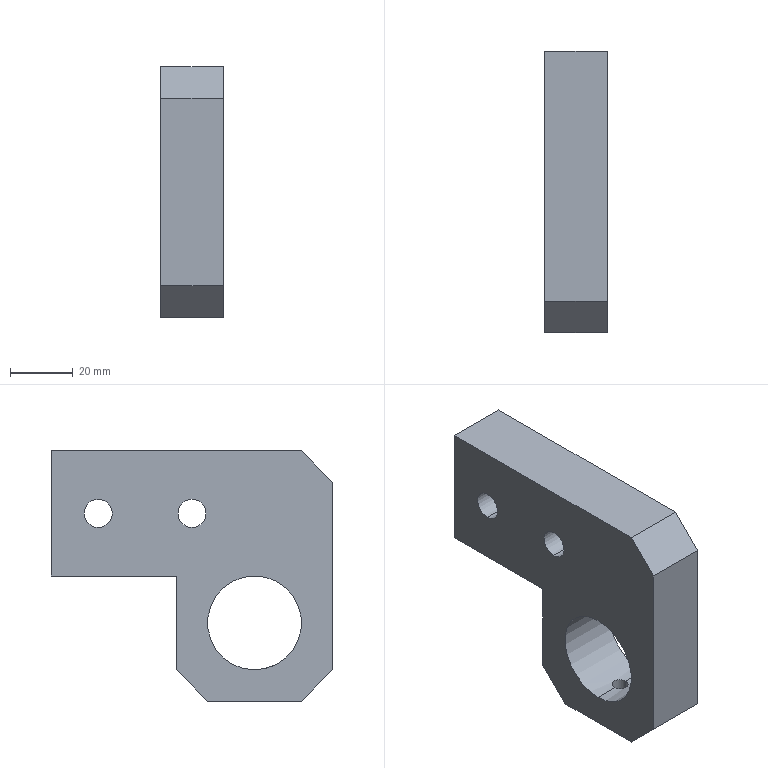Component | SolidWorks | UpperAxisBracket-1 | 1 solid | 19 faces | box 20 x 90 x 80 mm | volume 92121 mm3 | plane 11 | cylinder 8 | commonest cylinder face diameters 9 x4 5 x2 30 x2
build123d program:
from build123d import *

# Parameters (mm, degrees)
SKETCH1_R              = 15
BOSS_EXTRUDE1_DEPTH    = 20
SKETCH2_R              = 4.5
CUT_EXTRUDE1_DEPTH     = 123.066
CHAMFER1_SIZE          = 10
M6_TAPPED_HOLE1_REACH  = 124.066
M6_TAPPED_HOLE1_BORE_R = 2.5


with BuildPart() as part:
    # Sketch1 → Boss-Extrude1 (new body)
    with BuildSketch(Plane.XY):
        Polygon((0, 0), (0, 90), (80, 90), (80, 40), (40, 40), (40, 0), align=None)
        with Locations((55, 65)):
            Circle(SKETCH1_R, mode=Mode.SUBTRACT)
    extrude(amount=BOSS_EXTRUDE1_DEPTH)

    # Sketch2 → Cut-Extrude1 (cut, through all)
    with BuildSketch(Plane(origin=(0, 0, 0), x_dir=(-1, 0, 0), z_dir=(0, 0, -1))):
        with Locations((-20, 45)):
            Circle(SKETCH2_R)
        with Locations((-20, 15)):
            Circle(SKETCH2_R)
    extrude(amount=-CUT_EXTRUDE1_DEPTH, mode=Mode.SUBTRACT)

    # Chamfer1
    chamfer1_edges = [part.edges().sort_by_distance(p)[0] for p in [
        (0, 90, 10),
        (80, 90, 10),
        (80, 40, 10),
    ]]
    chamfer(chamfer1_edges, length=CHAMFER1_SIZE)

    # M6 Tapped Hole1 bore → M6 Tapped Hole1 (cut, up to next)
    with BuildSketch(Plane(origin=(80, 0, 0), x_dir=(0, 0, -1), z_dir=(1, 0, 0)), mode=Mode.PRIVATE) as m6_tapped_hole1_sk1:
        with Locations((-10, 65)):
            Circle(M6_TAPPED_HOLE1_BORE_R)
    m6_tapped_hole1_tool1 = extrude(m6_tapped_hole1_sk1.sketch, amount=-M6_TAPPED_HOLE1_REACH, mode=Mode.PRIVATE) & part.part
    add(m6_tapped_hole1_tool1.solids().sort_by_distance((80, 65, 10))[0], mode=Mode.SUBTRACT)


solid = part.part

# Placed as in the assembly
solid = solid.moved(Location((-5.532, -245.334, 1376.399), (180, -90, 0)))
STEP:
#1=COLOUR_RGB('',0.7922,0.8196,0.9333);
#2=FILL_AREA_STYLE_COLOUR('',#1);
#3=FILL_AREA_STYLE('',(#2));
#4=SURFACE_STYLE_FILL_AREA(#3);
#5=SURFACE_SIDE_STYLE('',(#4));
#6=SURFACE_STYLE_USAGE(.BOTH.,#5);
#7=PRESENTATION_STYLE_ASSIGNMENT((#6));
#8=CARTESIAN_POINT('',(-0.5131,-12.218,51.433));
#9=VERTEX_POINT('',#8);
#10=CARTESIAN_POINT('',(-0.7099,-12.218,51.433));
#11=VERTEX_POINT('',#10);
#12=CARTESIAN_POINT('',(-0.5131,-12.218,51.433));
#13=CARTESIAN_POINT('',(-0.5131,-12.211,51.433));
#14=CARTESIAN_POINT('',(-0.5137,-12.205,51.433));
#15=CARTESIAN_POINT('',(-0.5162,-12.192,51.434));
#16=CARTESIAN_POINT('',(-0.5181,-12.186,51.434));
#17=CARTESIAN_POINT('',(-0.5231,-12.174,51.435));
#18=CARTESIAN_POINT('',(-0.5261,-12.169,51.435));
#19=CARTESIAN_POINT('',(-0.5332,-12.158,51.436));
#20=CARTESIAN_POINT('',(-0.5374,-12.153,51.437));
#21=CARTESIAN_POINT('',(-0.551,-12.139,51.438));
#22=CARTESIAN_POINT('',(-0.5619,-12.132,51.439));
#23=CARTESIAN_POINT('',(-0.5797,-12.125,51.44));
#24=CARTESIAN_POINT('',(-0.5859,-12.123,51.441));
#25=CARTESIAN_POINT('',(-0.5986,-12.12,51.441));
#26=CARTESIAN_POINT('',(-0.605,-12.119,51.441));
#27=CARTESIAN_POINT('',(-0.6179,-12.119,51.441));
#28=CARTESIAN_POINT('',(-0.6244,-12.12,51.441));
#29=CARTESIAN_POINT('',(-0.637,-12.123,51.441));
#30=CARTESIAN_POINT('',(-0.6432,-12.124,51.44));
#31=CARTESIAN_POINT('',(-0.6551,-12.129,51.44));
#32=CARTESIAN_POINT('',(-0.6609,-12.132,51.439));
#33=CARTESIAN_POINT('',(-0.6715,-12.14,51.438));
#34=CARTESIAN_POINT('',(-0.6765,-12.144,51.438));
#35=CARTESIAN_POINT('',(-0.6857,-12.153,51.437));
#36=CARTESIAN_POINT('',(-0.6897,-12.158,51.436));
#37=CARTESIAN_POINT('',(-0.6969,-12.168,51.435));
#38=CARTESIAN_POINT('',(-0.6999,-12.174,51.435));
#39=CARTESIAN_POINT('',(-0.7049,-12.186,51.434));
#40=CARTESIAN_POINT('',(-0.7067,-12.192,51.434));
#41=CARTESIAN_POINT('',(-0.7093,-12.205,51.433));
#42=CARTESIAN_POINT('',(-0.7099,-12.211,51.433));
#43=CARTESIAN_POINT('',(-0.7099,-12.218,51.433));
#44=B_SPLINE_CURVE_WITH_KNOTS('',3,(#12,#13,#14,#15,#16,#17,#18,#19,#20,#21,#22,#23,#24,#25,#26,#27,#28,#29,#30,#31,#32,#33,#34,#35,#36,#37,#38,#39,#40,#41,#42,#43),.UNSPECIFIED.,.F.,.F.,(4,2,2,2,2,2,2,2,2,2,2,2,2,2,2,4),(0.,0.0004894,0.0009787,0.001468,0.001957,0.002936,0.003426,0.003915,0.004404,0.004894,0.005383,0.005872,0.006362,0.006851,0.00734,0.00783),.UNSPECIFIED.);
#45=EDGE_CURVE('',#9,#11,#44,.T.);
#46=ORIENTED_EDGE('',*,*,#45,.T.);
#47=CARTESIAN_POINT('',(-0.7099,-12.218,51.039));
#48=VERTEX_POINT('',#47);
#49=CARTESIAN_POINT('',(-0.7099,-12.218,51.039));
#50=DIRECTION('',(-0.,0.,-1.));
#51=VECTOR('',#50,39.37);
#52=LINE('',#49,#51);
#53=EDGE_CURVE('',#11,#48,#52,.T.);
#54=ORIENTED_EDGE('',*,*,#53,.T.);
#55=CARTESIAN_POINT('',(-0.5131,-12.218,51.039));
#56=VERTEX_POINT('',#55);
#57=CARTESIAN_POINT('',(-0.6115,-12.218,51.039));
#58=DIRECTION('',(-0.,0.,-1.));
#59=DIRECTION('',(1.,0.,0.));
#60=AXIS2_PLACEMENT_3D('',#57,#58,#59);
#61=CIRCLE('',#60,0.09843);
#62=EDGE_CURVE('',#48,#56,#61,.T.);
#63=ORIENTED_EDGE('',*,*,#62,.T.);
#64=CARTESIAN_POINT('',(-0.5131,-12.218,51.039));
#65=DIRECTION('',(-0.,0.,-1.));
#66=VECTOR('',#65,39.37);
#67=LINE('',#64,#66);
#68=EDGE_CURVE('',#9,#56,#67,.T.);
#69=ORIENTED_EDGE('',*,*,#68,.F.);
#70=EDGE_LOOP('',(#46,#54,#63,#69));
#71=FACE_OUTER_BOUND('',#70,.T.);
#72=CARTESIAN_POINT('',(-0.6115,-12.218,51.039));
#73=DIRECTION('',(-0.,0.,-1.));
#74=DIRECTION('',(1.,0.,0.));
#75=AXIS2_PLACEMENT_3D('',#72,#73,#74);
#76=CYLINDRICAL_SURFACE('',#75,0.09843);
#77=ADVANCED_FACE('',(#71),#76,.F.);
#78=CARTESIAN_POINT('',(-1.005,-10.249,53.224));
#79=VERTEX_POINT('',#78);
#80=CARTESIAN_POINT('',(-1.005,-10.249,53.579));
#81=VERTEX_POINT('',#80);
#82=CARTESIAN_POINT('',(-1.005,-10.249,53.402));
#83=DIRECTION('',(1.,0.,-0.));
#84=DIRECTION('',(0.,0.,1.));
#85=AXIS2_PLACEMENT_3D('',#82,#83,#84);
#86=CIRCLE('',#85,0.1772);
#87=EDGE_CURVE('',#79,#81,#86,.T.);
#88=ORIENTED_EDGE('',*,*,#87,.F.);
#89=CARTESIAN_POINT('',(-0.2178,-10.249,53.224));
#90=VERTEX_POINT('',#89);
#91=CARTESIAN_POINT('',(-1.005,-10.249,53.224));
#92=DIRECTION('',(1.,0.,-0.));
#93=VECTOR('',#92,39.37);
#94=LINE('',#91,#93);
#95=EDGE_CURVE('',#79,#90,#94,.T.);
#96=ORIENTED_EDGE('',*,*,#95,.T.);
#97=CARTESIAN_POINT('',(-0.2178,-10.249,53.579));
#98=VERTEX_POINT('',#97);
#99=CARTESIAN_POINT('',(-0.2178,-10.249,53.402));
#100=DIRECTION('',(1.,0.,-0.));
#101=DIRECTION('',(0.,0.,1.));
#102=AXIS2_PLACEMENT_3D('',#99,#100,#101);
#103=CIRCLE('',#102,0.1772);
#104=EDGE_CURVE('',#90,#98,#103,.T.);
#105=ORIENTED_EDGE('',*,*,#104,.T.);
#106=CARTESIAN_POINT('',(-1.005,-10.249,53.579));
#107=DIRECTION('',(1.,0.,-0.));
#108=VECTOR('',#107,39.37);
#109=LINE('',#106,#108);
#110=EDGE_CURVE('',#81,#98,#109,.T.);
#111=ORIENTED_EDGE('',*,*,#110,.F.);
#112=EDGE_LOOP('',(#88,#96,#105,#111));
#113=FACE_OUTER_BOUND('',#112,.T.);
#114=CARTESIAN_POINT('',(-1.005,-10.249,53.402));
#115=DIRECTION('',(1.,0.,-0.));
#116=DIRECTION('',(0.,0.,1.));
#117=AXIS2_PLACEMENT_3D('',#114,#115,#116);
#118=CYLINDRICAL_SURFACE('',#117,0.1772);
#119=ADVANCED_FACE('',(#113),#118,.F.);
#120=CARTESIAN_POINT('',(-1.005,-11.43,53.224));
#121=VERTEX_POINT('',#120);
#122=CARTESIAN_POINT('',(-1.005,-11.43,53.579));
#123=VERTEX_POINT('',#122);
#124=CARTESIAN_POINT('',(-1.005,-11.43,53.402));
#125=DIRECTION('',(1.,0.,-0.));
#126=DIRECTION('',(0.,0.,1.));
#127=AXIS2_PLACEMENT_3D('',#124,#125,#126);
#128=CIRCLE('',#127,0.1772);
#129=EDGE_CURVE('',#121,#123,#128,.T.);
#130=ORIENTED_EDGE('',*,*,#129,.F.);
#131=CARTESIAN_POINT('',(-0.2178,-11.43,53.224));
#132=VERTEX_POINT('',#131);
#133=CARTESIAN_POINT('',(-1.005,-11.43,53.224));
#134=DIRECTION('',(1.,0.,-0.));
#135=VECTOR('',#134,39.37);
#136=LINE('',#133,#135);
#137=EDGE_CURVE('',#121,#132,#136,.T.);
#138=ORIENTED_EDGE('',*,*,#137,.T.);
#139=CARTESIAN_POINT('',(-0.2178,-11.43,53.579));
#140=VERTEX_POINT('',#139);
#141=CARTESIAN_POINT('',(-0.2178,-11.43,53.402));
#142=DIRECTION('',(1.,0.,-0.));
#143=DIRECTION('',(0.,0.,1.));
#144=AXIS2_PLACEMENT_3D('',#141,#142,#143);
#145=CIRCLE('',#144,0.1772);
#146=EDGE_CURVE('',#132,#140,#145,.T.);
#147=ORIENTED_EDGE('',*,*,#146,.T.);
#148=CARTESIAN_POINT('',(-1.005,-11.43,53.579));
#149=DIRECTION('',(1.,0.,-0.));
#150=VECTOR('',#149,39.37);
#151=LINE('',#148,#150);
#152=EDGE_CURVE('',#123,#140,#151,.T.);
#153=ORIENTED_EDGE('',*,*,#152,.F.);
#154=EDGE_LOOP('',(#130,#138,#147,#153));
#155=FACE_OUTER_BOUND('',#154,.T.);
#156=CARTESIAN_POINT('',(-1.005,-11.43,53.402));
#157=DIRECTION('',(1.,0.,-0.));
#158=DIRECTION('',(0.,0.,1.));
#159=AXIS2_PLACEMENT_3D('',#156,#157,#158);
#160=CYLINDRICAL_SURFACE('',#159,0.1772);
#161=ADVANCED_FACE('',(#155),#160,.F.);
#162=CARTESIAN_POINT('',(-1.005,-12.218,52.614));
#163=VERTEX_POINT('',#162);
#164=CARTESIAN_POINT('',(-1.005,-12.218,51.433));
#165=VERTEX_POINT('',#164);
#166=CARTESIAN_POINT('',(-1.005,-12.218,52.024));
#167=DIRECTION('',(-1.,-0.,0.));
#168=DIRECTION('',(-0.,0.,-1.));
#169=AXIS2_PLACEMENT_3D('',#166,#167,#168);
#170=CIRCLE('',#169,0.5906);
#171=EDGE_CURVE('',#163,#165,#170,.T.);
#172=ORIENTED_EDGE('',*,*,#171,.T.);
#173=CARTESIAN_POINT('',(-1.005,-12.218,51.433));
#174=DIRECTION('',(1.,0.,-0.));
#175=VECTOR('',#174,39.37);
#176=LINE('',#173,#175);
#177=EDGE_CURVE('',#165,#11,#176,.T.);
#178=ORIENTED_EDGE('',*,*,#177,.T.);
#179=ORIENTED_EDGE('',*,*,#45,.F.);
#180=CARTESIAN_POINT('',(-0.2178,-12.218,51.433));
#181=VERTEX_POINT('',#180);
#182=CARTESIAN_POINT('',(-1.005,-12.218,51.433));
#183=DIRECTION('',(1.,0.,-0.));
#184=VECTOR('',#183,39.37);
#185=LINE('',#182,#184);
#186=EDGE_CURVE('',#9,#181,#185,.T.);
#187=ORIENTED_EDGE('',*,*,#186,.T.);
#188=CARTESIAN_POINT('',(-0.2178,-12.218,52.614));
#189=VERTEX_POINT('',#188);
#190=CARTESIAN_POINT('',(-0.2178,-12.218,52.024));
#191=DIRECTION('',(-1.,-0.,0.));
#192=DIRECTION('',(-0.,0.,-1.));
#193=AXIS2_PLACEMENT_3D('',#190,#191,#192);
#194=CIRCLE('',#193,0.5906);
#195=EDGE_CURVE('',#189,#181,#194,.T.);
#196=ORIENTED_EDGE('',*,*,#195,.F.);
#197=CARTESIAN_POINT('',(-1.005,-12.218,52.614));
#198=DIRECTION('',(1.,0.,-0.));
#199=VECTOR('',#198,39.37);
#200=LINE('',#197,#199);
#201=EDGE_CURVE('',#163,#189,#200,.T.);
#202=ORIENTED_EDGE('',*,*,#201,.F.);
#203=EDGE_LOOP('',(#172,#178,#179,#187,#196,#202));
#204=FACE_OUTER_BOUND('',#203,.T.);
#205=CARTESIAN_POINT('',(-1.005,-12.218,52.024));
#206=DIRECTION('',(1.,0.,-0.));
#207=DIRECTION('',(0.,0.,1.));
#208=AXIS2_PLACEMENT_3D('',#205,#206,#207);
#209=CYLINDRICAL_SURFACE('',#208,0.5906);
#210=ADVANCED_FACE('',(#204),#209,.F.);
#211=CARTESIAN_POINT('',(-1.005,-10.249,53.402));
#212=DIRECTION('',(1.,0.,-0.));
#213=DIRECTION('',(0.,0.,1.));
#214=AXIS2_PLACEMENT_3D('',#211,#212,#213);
#215=CIRCLE('',#214,0.1772);
#216=EDGE_CURVE('',#81,#79,#215,.T.);
#217=ORIENTED_EDGE('',*,*,#216,.T.);
#218=ORIENTED_EDGE('',*,*,#87,.T.);
#219=EDGE_LOOP('',(#217,#218));
#220=FACE_BOUND('',#219,.T.);
#221=CARTESIAN_POINT('',(-1.005,-11.43,53.402));
#222=DIRECTION('',(1.,0.,-0.));
#223=DIRECTION('',(0.,0.,1.));
#224=AXIS2_PLACEMENT_3D('',#221,#222,#223);
#225=CIRCLE('',#224,0.1772);
#226=EDGE_CURVE('',#123,#121,#225,.T.);
#227=ORIENTED_EDGE('',*,*,#226,.T.);
#228=ORIENTED_EDGE('',*,*,#129,.T.);
#229=EDGE_LOOP('',(#227,#228));
#230=FACE_BOUND('',#229,.T.);
#231=CARTESIAN_POINT('',(-1.005,-11.234,52.614));
#232=VERTEX_POINT('',#231);
#233=CARTESIAN_POINT('',(-1.005,-11.234,51.433));
#234=VERTEX_POINT('',#233);
#235=CARTESIAN_POINT('',(-1.005,-11.234,51.039));
#236=DIRECTION('',(-0.,0.,-1.));
#237=VECTOR('',#236,39.37);
#238=LINE('',#235,#237);
#239=EDGE_CURVE('',#232,#234,#238,.T.);
#240=ORIENTED_EDGE('',*,*,#239,.T.);
#241=CARTESIAN_POINT('',(-1.005,-11.627,51.039));
#242=VERTEX_POINT('',#241);
#243=CARTESIAN_POINT('',(-1.005,-11.627,51.039));
#244=DIRECTION('',(-0.,-0.7071,-0.7071));
#245=VECTOR('',#244,39.37);
#246=LINE('',#243,#245);
#247=EDGE_CURVE('',#234,#242,#246,.T.);
#248=ORIENTED_EDGE('',*,*,#247,.T.);
#249=CARTESIAN_POINT('',(-1.005,-12.808,51.039));
#250=VERTEX_POINT('',#249);
#251=CARTESIAN_POINT('',(-1.005,-13.202,51.039));
#252=DIRECTION('',(0.,-1.,-0.));
#253=VECTOR('',#252,39.37);
#254=LINE('',#251,#253);
#255=EDGE_CURVE('',#242,#250,#254,.T.);
#256=ORIENTED_EDGE('',*,*,#255,.T.);
#257=CARTESIAN_POINT('',(-1.005,-13.202,51.433));
#258=VERTEX_POINT('',#257);
#259=CARTESIAN_POINT('',(-1.005,-13.202,51.433));
#260=DIRECTION('',(0.,-0.7071,0.7071));
#261=VECTOR('',#260,39.37);
#262=LINE('',#259,#261);
#263=EDGE_CURVE('',#250,#258,#262,.T.);
#264=ORIENTED_EDGE('',*,*,#263,.T.);
#265=CARTESIAN_POINT('',(-1.005,-13.202,53.795));
#266=VERTEX_POINT('',#265);
#267=CARTESIAN_POINT('',(-1.005,-13.202,54.189));
#268=DIRECTION('',(0.,-0.,1.));
#269=VECTOR('',#268,39.37);
#270=LINE('',#267,#269);
#271=EDGE_CURVE('',#258,#266,#270,.T.);
#272=ORIENTED_EDGE('',*,*,#271,.T.);
#273=CARTESIAN_POINT('',(-1.005,-12.808,54.189));
#274=VERTEX_POINT('',#273);
#275=CARTESIAN_POINT('',(-1.005,-12.808,54.189));
#276=DIRECTION('',(0.,0.7071,0.7071));
#277=VECTOR('',#276,39.37);
#278=LINE('',#275,#277);
#279=EDGE_CURVE('',#266,#274,#278,.T.);
#280=ORIENTED_EDGE('',*,*,#279,.T.);
#281=CARTESIAN_POINT('',(-1.005,-9.659,54.189));
#282=VERTEX_POINT('',#281);
#283=CARTESIAN_POINT('',(-1.005,-9.659,54.189));
#284=DIRECTION('',(-0.,1.,0.));
#285=VECTOR('',#284,39.37);
#286=LINE('',#283,#285);
#287=EDGE_CURVE('',#274,#282,#286,.T.);
#288=ORIENTED_EDGE('',*,*,#287,.T.);
#289=CARTESIAN_POINT('',(-1.005,-9.659,52.614));
#290=VERTEX_POINT('',#289);
#291=CARTESIAN_POINT('',(-1.005,-9.659,52.614));
#292=DIRECTION('',(-0.,0.,-1.));
#293=VECTOR('',#292,39.37);
#294=LINE('',#291,#293);
#295=EDGE_CURVE('',#282,#290,#294,.T.);
#296=ORIENTED_EDGE('',*,*,#295,.T.);
#297=CARTESIAN_POINT('',(-1.005,-11.234,52.614));
#298=DIRECTION('',(0.,-1.,-0.));
#299=VECTOR('',#298,39.37);
#300=LINE('',#297,#299);
#301=EDGE_CURVE('',#290,#232,#300,.T.);
#302=ORIENTED_EDGE('',*,*,#301,.T.);
#303=EDGE_LOOP('',(#240,#248,#256,#264,#272,#280,#288,#296,#302));
#304=FACE_OUTER_BOUND('',#303,.T.);
#305=ORIENTED_EDGE('',*,*,#171,.F.);
#306=CARTESIAN_POINT('',(-1.005,-12.218,52.024));
#307=DIRECTION('',(-1.,-0.,0.));
#308=DIRECTION('',(-0.,0.,-1.));
#309=AXIS2_PLACEMENT_3D('',#306,#307,#308);
#310=CIRCLE('',#309,0.5906);
#311=EDGE_CURVE('',#165,#163,#310,.T.);
#312=ORIENTED_EDGE('',*,*,#311,.F.);
#313=EDGE_LOOP('',(#305,#312));
#314=FACE_BOUND('',#313,.T.);
#315=CARTESIAN_POINT('',(-1.005,-9.659,54.189));
#316=DIRECTION('',(1.,0.,-0.));
#317=DIRECTION('',(0.,-0.,1.));
#318=AXIS2_PLACEMENT_3D('',#315,#316,#317);
#319=PLANE('',#318);
#320=ADVANCED_FACE('',(#220,#230,#304,#314),#319,.F.);
#321=CARTESIAN_POINT('',(-0.2178,-10.249,53.402));
#322=DIRECTION('',(1.,0.,-0.));
#323=DIRECTION('',(0.,0.,1.));
#324=AXIS2_PLACEMENT_3D('',#321,#322,#323);
#325=CIRCLE('',#324,0.1772);
#326=EDGE_CURVE('',#98,#90,#325,.T.);
#327=ORIENTED_EDGE('',*,*,#326,.F.);
#328=ORIENTED_EDGE('',*,*,#104,.F.);
#329=EDGE_LOOP('',(#327,#328));
#330=FACE_BOUND('',#329,.T.);
#331=CARTESIAN_POINT('',(-0.2178,-11.43,53.402));
#332=DIRECTION('',(1.,0.,-0.));
#333=DIRECTION('',(0.,0.,1.));
#334=AXIS2_PLACEMENT_3D('',#331,#332,#333);
#335=CIRCLE('',#334,0.1772);
#336=EDGE_CURVE('',#140,#132,#335,.T.);
#337=ORIENTED_EDGE('',*,*,#336,.F.);
#338=ORIENTED_EDGE('',*,*,#146,.F.);
#339=EDGE_LOOP('',(#337,#338));
#340=FACE_BOUND('',#339,.T.);
#341=CARTESIAN_POINT('',(-0.2178,-11.627,51.039));
#342=VERTEX_POINT('',#341);
#343=CARTESIAN_POINT('',(-0.2178,-12.808,51.039));
#344=VERTEX_POINT('',#343);
#345=CARTESIAN_POINT('',(-0.2178,-13.202,51.039));
#346=DIRECTION('',(0.,-1.,-0.));
#347=VECTOR('',#346,39.37);
#348=LINE('',#345,#347);
#349=EDGE_CURVE('',#342,#344,#348,.T.);
#350=ORIENTED_EDGE('',*,*,#349,.F.);
#351=CARTESIAN_POINT('',(-0.2178,-11.234,51.433));
#352=VERTEX_POINT('',#351);
#353=CARTESIAN_POINT('',(-0.2178,-9.068,53.598));
#354=DIRECTION('',(0.,0.7071,0.7071));
#355=VECTOR('',#354,39.37);
#356=LINE('',#353,#355);
#357=EDGE_CURVE('',#342,#352,#356,.T.);
#358=ORIENTED_EDGE('',*,*,#357,.T.);
#359=CARTESIAN_POINT('',(-0.2178,-11.234,52.614));
#360=VERTEX_POINT('',#359);
#361=CARTESIAN_POINT('',(-0.2178,-11.234,51.039));
#362=DIRECTION('',(-0.,0.,-1.));
#363=VECTOR('',#362,39.37);
#364=LINE('',#361,#363);
#365=EDGE_CURVE('',#360,#352,#364,.T.);
#366=ORIENTED_EDGE('',*,*,#365,.F.);
#367=CARTESIAN_POINT('',(-0.2178,-9.659,52.614));
#368=VERTEX_POINT('',#367);
#369=CARTESIAN_POINT('',(-0.2178,-11.234,52.614));
#370=DIRECTION('',(0.,-1.,-0.));
#371=VECTOR('',#370,39.37);
#372=LINE('',#369,#371);
#373=EDGE_CURVE('',#368,#360,#372,.T.);
#374=ORIENTED_EDGE('',*,*,#373,.F.);
#375=CARTESIAN_POINT('',(-0.2178,-9.659,54.189));
#376=VERTEX_POINT('',#375);
#377=CARTESIAN_POINT('',(-0.2178,-9.659,52.614));
#378=DIRECTION('',(-0.,0.,-1.));
#379=VECTOR('',#378,39.37);
#380=LINE('',#377,#379);
#381=EDGE_CURVE('',#376,#368,#380,.T.);
#382=ORIENTED_EDGE('',*,*,#381,.F.);
#383=CARTESIAN_POINT('',(-0.2178,-12.808,54.189));
#384=VERTEX_POINT('',#383);
#385=CARTESIAN_POINT('',(-0.2178,-9.659,54.189));
#386=DIRECTION('',(-0.,1.,0.));
#387=VECTOR('',#386,39.37);
#388=LINE('',#385,#387);
#389=EDGE_CURVE('',#384,#376,#388,.T.);
#390=ORIENTED_EDGE('',*,*,#389,.F.);
#391=CARTESIAN_POINT('',(-0.2178,-13.202,53.795));
#392=VERTEX_POINT('',#391);
#393=CARTESIAN_POINT('',(-0.2178,-11.234,55.764));
#394=DIRECTION('',(-0.,-0.7071,-0.7071));
#395=VECTOR('',#394,39.37);
#396=LINE('',#393,#395);
#397=EDGE_CURVE('',#384,#392,#396,.T.);
#398=ORIENTED_EDGE('',*,*,#397,.T.);
#399=CARTESIAN_POINT('',(-0.2178,-13.202,51.433));
#400=VERTEX_POINT('',#399);
#401=CARTESIAN_POINT('',(-0.2178,-13.202,54.189));
#402=DIRECTION('',(0.,-0.,1.));
#403=VECTOR('',#402,39.37);
#404=LINE('',#401,#403);
#405=EDGE_CURVE('',#400,#392,#404,.T.);
#406=ORIENTED_EDGE('',*,*,#405,.F.);
#407=CARTESIAN_POINT('',(-0.2178,-12.808,51.039));
#408=DIRECTION('',(-0.,0.7071,-0.7071));
#409=VECTOR('',#408,39.37);
#410=LINE('',#407,#409);
#411=EDGE_CURVE('',#400,#344,#410,.T.);
#412=ORIENTED_EDGE('',*,*,#411,.T.);
#413=EDGE_LOOP('',(#350,#358,#366,#374,#382,#390,#398,#406,#412));
#414=FACE_OUTER_BOUND('',#413,.T.);
#415=ORIENTED_EDGE('',*,*,#195,.T.);
#416=CARTESIAN_POINT('',(-0.2178,-12.218,52.024));
#417=DIRECTION('',(-1.,-0.,0.));
#418=DIRECTION('',(-0.,0.,-1.));
#419=AXIS2_PLACEMENT_3D('',#416,#417,#418);
#420=CIRCLE('',#419,0.5906);
#421=EDGE_CURVE('',#181,#189,#420,.T.);
#422=ORIENTED_EDGE('',*,*,#421,.T.);
#423=EDGE_LOOP('',(#415,#422));
#424=FACE_BOUND('',#423,.T.);
#425=CARTESIAN_POINT('',(-0.2178,-9.659,54.189));
#426=DIRECTION('',(1.,0.,-0.));
#427=DIRECTION('',(0.,-0.,1.));
#428=AXIS2_PLACEMENT_3D('',#425,#426,#427);
#429=PLANE('',#428);
#430=ADVANCED_FACE('',(#330,#340,#414,#424),#429,.T.);
#431=ORIENTED_EDGE('',*,*,#381,.T.);
#432=CARTESIAN_POINT('',(-1.005,-9.659,52.614));
#433=DIRECTION('',(1.,0.,-0.));
#434=VECTOR('',#433,39.37);
#435=LINE('',#432,#434);
#436=EDGE_CURVE('',#290,#368,#435,.T.);
#437=ORIENTED_EDGE('',*,*,#436,.F.);
#438=ORIENTED_EDGE('',*,*,#295,.F.);
#439=CARTESIAN_POINT('',(-1.005,-9.659,54.189));
#440=DIRECTION('',(1.,0.,-0.));
#441=VECTOR('',#440,39.37);
#442=LINE('',#439,#441);
#443=EDGE_CURVE('',#282,#376,#442,.T.);
#444=ORIENTED_EDGE('',*,*,#443,.T.);
#445=EDGE_LOOP('',(#431,#437,#438,#444));
#446=FACE_OUTER_BOUND('',#445,.T.);
#447=CARTESIAN_POINT('',(-1.005,-9.659,52.614));
#448=DIRECTION('',(0.,-1.,-0.));
#449=DIRECTION('',(0.,-0.,1.));
#450=AXIS2_PLACEMENT_3D('',#447,#448,#449);
#451=PLANE('',#450);
#452=ADVANCED_FACE('',(#446),#451,.F.);
#453=ORIENTED_EDGE('',*,*,#373,.T.);
#454=CARTESIAN_POINT('',(-1.005,-11.234,52.614));
#455=DIRECTION('',(1.,0.,-0.));
#456=VECTOR('',#455,39.37);
#457=LINE('',#454,#456);
#458=EDGE_CURVE('',#232,#360,#457,.T.);
#459=ORIENTED_EDGE('',*,*,#458,.F.);
#460=ORIENTED_EDGE('',*,*,#301,.F.);
#461=ORIENTED_EDGE('',*,*,#436,.T.);
#462=EDGE_LOOP('',(#453,#459,#460,#461));
#463=FACE_OUTER_BOUND('',#462,.T.);
#464=CARTESIAN_POINT('',(-1.005,-11.234,52.614));
#465=DIRECTION('',(0.,-0.,1.));
#466=DIRECTION('',(-1.,-0.,0.));
#467=AXIS2_PLACEMENT_3D('',#464,#465,#466);
#468=PLANE('',#467);
#469=ADVANCED_FACE('',(#463),#468,.F.);
#470=ORIENTED_EDGE('',*,*,#365,.T.);
#471=CARTESIAN_POINT('',(-1.005,-11.234,51.433));
#472=DIRECTION('',(-1.,-0.,0.));
#473=VECTOR('',#472,39.37);
#474=LINE('',#471,#473);
#475=EDGE_CURVE('',#352,#234,#474,.T.);
#476=ORIENTED_EDGE('',*,*,#475,.T.);
#477=ORIENTED_EDGE('',*,*,#239,.F.);
#478=ORIENTED_EDGE('',*,*,#458,.T.);
#479=EDGE_LOOP('',(#470,#476,#477,#478));
#480=FACE_OUTER_BOUND('',#479,.T.);
#481=CARTESIAN_POINT('',(-1.005,-11.234,51.039));
#482=DIRECTION('',(0.,-1.,-0.));
#483=DIRECTION('',(-1.,-0.,0.));
#484=AXIS2_PLACEMENT_3D('',#481,#482,#483);
#485=PLANE('',#484);
#486=ADVANCED_FACE('',(#480),#485,.F.);
#487=CARTESIAN_POINT('',(-0.6115,-12.218,51.039));
#488=DIRECTION('',(-0.,0.,-1.));
#489=DIRECTION('',(1.,0.,0.));
#490=AXIS2_PLACEMENT_3D('',#487,#488,#489);
#491=CIRCLE('',#490,0.09843);
#492=EDGE_CURVE('',#56,#48,#491,.T.);
#493=ORIENTED_EDGE('',*,*,#492,.F.);
#494=ORIENTED_EDGE('',*,*,#62,.F.);
#495=EDGE_LOOP('',(#493,#494));
#496=FACE_BOUND('',#495,.T.);
#497=ORIENTED_EDGE('',*,*,#255,.F.);
#498=CARTESIAN_POINT('',(-1.005,-11.627,51.039));
#499=DIRECTION('',(1.,0.,-0.));
#500=VECTOR('',#499,39.37);
#501=LINE('',#498,#500);
#502=EDGE_CURVE('',#242,#342,#501,.T.);
#503=ORIENTED_EDGE('',*,*,#502,.T.);
#504=ORIENTED_EDGE('',*,*,#349,.T.);
#505=CARTESIAN_POINT('',(-1.005,-12.808,51.039));
#506=DIRECTION('',(-1.,-0.,0.));
#507=VECTOR('',#506,39.37);
#508=LINE('',#505,#507);
#509=EDGE_CURVE('',#344,#250,#508,.T.);
#510=ORIENTED_EDGE('',*,*,#509,.T.);
#511=EDGE_LOOP('',(#497,#503,#504,#510));
#512=FACE_OUTER_BOUND('',#511,.T.);
#513=CARTESIAN_POINT('',(-1.005,-13.202,51.039));
#514=DIRECTION('',(0.,-0.,1.));
#515=DIRECTION('',(-1.,-0.,0.));
#516=AXIS2_PLACEMENT_3D('',#513,#514,#515);
#517=PLANE('',#516);
#518=ADVANCED_FACE('',(#496,#512),#517,.F.);
#519=ORIENTED_EDGE('',*,*,#405,.T.);
#520=CARTESIAN_POINT('',(-1.005,-13.202,53.795));
#521=DIRECTION('',(-1.,-0.,0.));
#522=VECTOR('',#521,39.37);
#523=LINE('',#520,#522);
#524=EDGE_CURVE('',#392,#266,#523,.T.);
#525=ORIENTED_EDGE('',*,*,#524,.T.);
#526=ORIENTED_EDGE('',*,*,#271,.F.);
#527=CARTESIAN_POINT('',(-1.005,-13.202,51.433));
#528=DIRECTION('',(1.,0.,-0.));
#529=VECTOR('',#528,39.37);
#530=LINE('',#527,#529);
#531=EDGE_CURVE('',#258,#400,#530,.T.);
#532=ORIENTED_EDGE('',*,*,#531,.T.);
#533=EDGE_LOOP('',(#519,#525,#526,#532));
#534=FACE_OUTER_BOUND('',#533,.T.);
#535=CARTESIAN_POINT('',(-1.005,-13.202,54.189));
#536=DIRECTION('',(-0.,1.,0.));
#537=DIRECTION('',(1.,0.,-0.));
#538=AXIS2_PLACEMENT_3D('',#535,#536,#537);
#539=PLANE('',#538);
#540=ADVANCED_FACE('',(#534),#539,.F.);
#541=ORIENTED_EDGE('',*,*,#287,.F.);
#542=CARTESIAN_POINT('',(-1.005,-12.808,54.189));
#543=DIRECTION('',(1.,0.,-0.));
#544=VECTOR('',#543,39.37);
#545=LINE('',#542,#544);
#546=EDGE_CURVE('',#274,#384,#545,.T.);
#547=ORIENTED_EDGE('',*,*,#546,.T.);
#548=ORIENTED_EDGE('',*,*,#389,.T.);
#549=ORIENTED_EDGE('',*,*,#443,.F.);
#550=EDGE_LOOP('',(#541,#547,#548,#549));
#551=FACE_OUTER_BOUND('',#550,.T.);
#552=CARTESIAN_POINT('',(-1.005,-9.659,54.189));
#553=DIRECTION('',(-0.,0.,-1.));
#554=DIRECTION('',(1.,0.,-0.));
#555=AXIS2_PLACEMENT_3D('',#552,#553,#554);
#556=PLANE('',#555);
#557=ADVANCED_FACE('',(#551),#556,.F.);
#558=ORIENTED_EDGE('',*,*,#177,.F.);
#559=ORIENTED_EDGE('',*,*,#311,.T.);
#560=ORIENTED_EDGE('',*,*,#201,.T.);
#561=ORIENTED_EDGE('',*,*,#421,.F.);
#562=ORIENTED_EDGE('',*,*,#186,.F.);
#563=CARTESIAN_POINT('',(-0.7099,-12.218,51.433));
#564=CARTESIAN_POINT('',(-0.7099,-12.231,51.433));
#565=CARTESIAN_POINT('',(-0.7073,-12.244,51.433));
#566=CARTESIAN_POINT('',(-0.7,-12.261,51.435));
#567=CARTESIAN_POINT('',(-0.6969,-12.267,51.435));
#568=CARTESIAN_POINT('',(-0.6897,-12.278,51.436));
#569=CARTESIAN_POINT('',(-0.6857,-12.283,51.437));
#570=CARTESIAN_POINT('',(-0.6766,-12.292,51.438));
#571=CARTESIAN_POINT('',(-0.6715,-12.296,51.438));
#572=CARTESIAN_POINT('',(-0.6609,-12.303,51.439));
#573=CARTESIAN_POINT('',(-0.6552,-12.306,51.44));
#574=CARTESIAN_POINT('',(-0.6433,-12.311,51.44));
#575=CARTESIAN_POINT('',(-0.6371,-12.313,51.441));
#576=CARTESIAN_POINT('',(-0.6245,-12.316,51.441));
#577=CARTESIAN_POINT('',(-0.618,-12.316,51.441));
#578=CARTESIAN_POINT('',(-0.605,-12.316,51.441));
#579=CARTESIAN_POINT('',(-0.5986,-12.316,51.441));
#580=CARTESIAN_POINT('',(-0.586,-12.313,51.441));
#581=CARTESIAN_POINT('',(-0.5798,-12.311,51.44));
#582=CARTESIAN_POINT('',(-0.5679,-12.306,51.44));
#583=CARTESIAN_POINT('',(-0.5622,-12.303,51.439));
#584=CARTESIAN_POINT('',(-0.5515,-12.296,51.438));
#585=CARTESIAN_POINT('',(-0.5465,-12.292,51.438));
#586=CARTESIAN_POINT('',(-0.5329,-12.278,51.436));
#587=CARTESIAN_POINT('',(-0.5255,-12.268,51.435));
#588=CARTESIAN_POINT('',(-0.5181,-12.25,51.434));
#589=CARTESIAN_POINT('',(-0.5162,-12.244,51.434));
#590=CARTESIAN_POINT('',(-0.5137,-12.231,51.433));
#591=CARTESIAN_POINT('',(-0.5131,-12.224,51.433));
#592=CARTESIAN_POINT('',(-0.5131,-12.218,51.433));
#593=B_SPLINE_CURVE_WITH_KNOTS('',3,(#563,#564,#565,#566,#567,#568,#569,#570,#571,#572,#573,#574,#575,#576,#577,#578,#579,#580,#581,#582,#583,#584,#585,#586,#587,#588,#589,#590,#591,#592),.UNSPECIFIED.,.F.,.F.,(4,2,2,2,2,2,2,2,2,2,2,2,2,2,4),(0.00783,0.008808,0.009298,0.009787,0.01028,0.01077,0.01125,0.01174,0.01223,0.01272,0.01321,0.0137,0.01468,0.01517,0.01566),.UNSPECIFIED.);
#594=EDGE_CURVE('',#11,#9,#593,.T.);
#595=ORIENTED_EDGE('',*,*,#594,.F.);
#596=EDGE_LOOP('',(#558,#559,#560,#561,#562,#595));
#597=FACE_OUTER_BOUND('',#596,.T.);
#598=CARTESIAN_POINT('',(-1.005,-12.218,52.024));
#599=DIRECTION('',(1.,0.,-0.));
#600=DIRECTION('',(0.,0.,1.));
#601=AXIS2_PLACEMENT_3D('',#598,#599,#600);
#602=CYLINDRICAL_SURFACE('',#601,0.5906);
#603=ADVANCED_FACE('',(#597),#602,.F.);
#604=ORIENTED_EDGE('',*,*,#137,.F.);
#605=ORIENTED_EDGE('',*,*,#226,.F.);
#606=ORIENTED_EDGE('',*,*,#152,.T.);
#607=ORIENTED_EDGE('',*,*,#336,.T.);
#608=EDGE_LOOP('',(#604,#605,#606,#607));
#609=FACE_OUTER_BOUND('',#608,.T.);
#610=CARTESIAN_POINT('',(-1.005,-11.43,53.402));
#611=DIRECTION('',(1.,0.,-0.));
#612=DIRECTION('',(0.,0.,1.));
#613=AXIS2_PLACEMENT_3D('',#610,#611,#612);
#614=CYLINDRICAL_SURFACE('',#613,0.1772);
#615=ADVANCED_FACE('',(#609),#614,.F.);
#616=ORIENTED_EDGE('',*,*,#95,.F.);
#617=ORIENTED_EDGE('',*,*,#216,.F.);
#618=ORIENTED_EDGE('',*,*,#110,.T.);
#619=ORIENTED_EDGE('',*,*,#326,.T.);
#620=EDGE_LOOP('',(#616,#617,#618,#619));
#621=FACE_OUTER_BOUND('',#620,.T.);
#622=CARTESIAN_POINT('',(-1.005,-10.249,53.402));
#623=DIRECTION('',(1.,0.,-0.));
#624=DIRECTION('',(0.,0.,1.));
#625=AXIS2_PLACEMENT_3D('',#622,#623,#624);
#626=CYLINDRICAL_SURFACE('',#625,0.1772);
#627=ADVANCED_FACE('',(#621),#626,.F.);
#628=ORIENTED_EDGE('',*,*,#247,.F.);
#629=ORIENTED_EDGE('',*,*,#475,.F.);
#630=ORIENTED_EDGE('',*,*,#357,.F.);
#631=ORIENTED_EDGE('',*,*,#502,.F.);
#632=EDGE_LOOP('',(#628,#629,#630,#631));
#633=FACE_OUTER_BOUND('',#632,.T.);
#634=CARTESIAN_POINT('',(-1.005,-11.627,51.039));
#635=DIRECTION('',(0.,-0.7071,0.7071));
#636=DIRECTION('',(1.,0.,-0.));
#637=AXIS2_PLACEMENT_3D('',#634,#635,#636);
#638=PLANE('',#637);
#639=ADVANCED_FACE('',(#633),#638,.F.);
#640=ORIENTED_EDGE('',*,*,#279,.F.);
#641=ORIENTED_EDGE('',*,*,#524,.F.);
#642=ORIENTED_EDGE('',*,*,#397,.F.);
#643=ORIENTED_EDGE('',*,*,#546,.F.);
#644=EDGE_LOOP('',(#640,#641,#642,#643));
#645=FACE_OUTER_BOUND('',#644,.T.);
#646=CARTESIAN_POINT('',(-1.005,-12.808,54.189));
#647=DIRECTION('',(-0.,0.7071,-0.7071));
#648=DIRECTION('',(1.,0.,-0.));
#649=AXIS2_PLACEMENT_3D('',#646,#647,#648);
#650=PLANE('',#649);
#651=ADVANCED_FACE('',(#645),#650,.F.);
#652=ORIENTED_EDGE('',*,*,#263,.F.);
#653=ORIENTED_EDGE('',*,*,#509,.F.);
#654=ORIENTED_EDGE('',*,*,#411,.F.);
#655=ORIENTED_EDGE('',*,*,#531,.F.);
#656=EDGE_LOOP('',(#652,#653,#654,#655));
#657=FACE_OUTER_BOUND('',#656,.T.);
#658=CARTESIAN_POINT('',(-1.005,-13.202,51.433));
#659=DIRECTION('',(0.,0.7071,0.7071));
#660=DIRECTION('',(1.,0.,-0.));
#661=AXIS2_PLACEMENT_3D('',#658,#659,#660);
#662=PLANE('',#661);
#663=ADVANCED_FACE('',(#657),#662,.F.);
#664=ORIENTED_EDGE('',*,*,#53,.F.);
#665=ORIENTED_EDGE('',*,*,#594,.T.);
#666=ORIENTED_EDGE('',*,*,#68,.T.);
#667=ORIENTED_EDGE('',*,*,#492,.T.);
#668=EDGE_LOOP('',(#664,#665,#666,#667));
#669=FACE_OUTER_BOUND('',#668,.T.);
#670=CARTESIAN_POINT('',(-0.6115,-12.218,51.039));
#671=DIRECTION('',(-0.,0.,-1.));
#672=DIRECTION('',(1.,0.,0.));
#673=AXIS2_PLACEMENT_3D('',#670,#671,#672);
#674=CYLINDRICAL_SURFACE('',#673,0.09843);
#675=ADVANCED_FACE('',(#669),#674,.F.);
#676=CLOSED_SHELL('',(#77,#119,#161,#210,#320,#430,#452,#469,#486,#518,#540,#557,#603,#615,#627,#639,#651,#663,#675));
#677=MANIFOLD_SOLID_BREP('',#676);
#678=STYLED_ITEM('',(#7),#677);
#679=PRESENTATION_LAYER_ASSIGNMENT('','',(#678));
#680=CARTESIAN_POINT('',(0.,0.,0.));
#681=DIRECTION('',(0.,0.,1.));
#682=DIRECTION('',(1.,0.,0.));
#683=AXIS2_PLACEMENT_3D('',#680,#681,#682);
#684=(LENGTH_UNIT()NAMED_UNIT(*)SI_UNIT($,.METRE.));
#685=LENGTH_MEASURE_WITH_UNIT(LENGTH_MEASURE(0.0254),#684);
#686=DIMENSIONAL_EXPONENTS(1.,0.,0.,0.,0.,0.,0.);
#687=(CONVERSION_BASED_UNIT('',#685)LENGTH_UNIT()NAMED_UNIT(#686));
#688=UNCERTAINTY_MEASURE_WITH_UNIT(LENGTH_MEASURE(0.00001),#687,'','');
#689=(NAMED_UNIT(*)PLANE_ANGLE_UNIT()SI_UNIT($,.RADIAN.));
#690=(NAMED_UNIT(*)SI_UNIT($,.STERADIAN.)SOLID_ANGLE_UNIT());
#691=(GEOMETRIC_REPRESENTATION_CONTEXT(3)GLOBAL_UNCERTAINTY_ASSIGNED_CONTEXT((#688))GLOBAL_UNIT_ASSIGNED_CONTEXT((#687,#689,#690))REPRESENTATION_CONTEXT('',''));
#692=ADVANCED_BREP_SHAPE_REPRESENTATION('',(#677,#683),#691);
#693=(LENGTH_UNIT()NAMED_UNIT(*)SI_UNIT($,.METRE.));
#694=LENGTH_MEASURE_WITH_UNIT(LENGTH_MEASURE(0.0254),#693);
#695=DIMENSIONAL_EXPONENTS(1.,0.,0.,0.,0.,0.,0.);
#696=(CONVERSION_BASED_UNIT('',#694)LENGTH_UNIT()NAMED_UNIT(#695));
#697=UNCERTAINTY_MEASURE_WITH_UNIT(LENGTH_MEASURE(0.00001),#696,'','');
#698=(NAMED_UNIT(*)PLANE_ANGLE_UNIT()SI_UNIT($,.RADIAN.));
#699=(NAMED_UNIT(*)SI_UNIT($,.STERADIAN.)SOLID_ANGLE_UNIT());
#700=(GEOMETRIC_REPRESENTATION_CONTEXT(3)GLOBAL_UNCERTAINTY_ASSIGNED_CONTEXT((#697))GLOBAL_UNIT_ASSIGNED_CONTEXT((#696,#698,#699))REPRESENTATION_CONTEXT('',''));
#701=MECHANICAL_DESIGN_GEOMETRIC_PRESENTATION_REPRESENTATION('',(#678),#700);